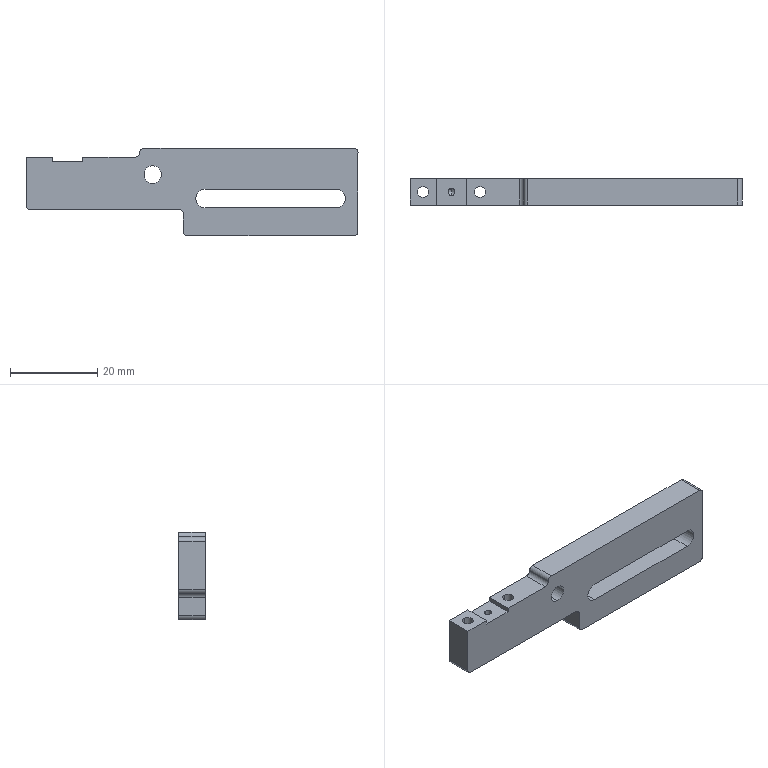Component | SolidWorks | F01AE00111-A5212-1 | 1 solid | 38 faces | volume 6363 mm3 | cylinder 19 | plane 15 | cone 4 | commonest cylinder face diameters 2 x7 2.5 x6 4 x2 1.6 x2 4.3 x2